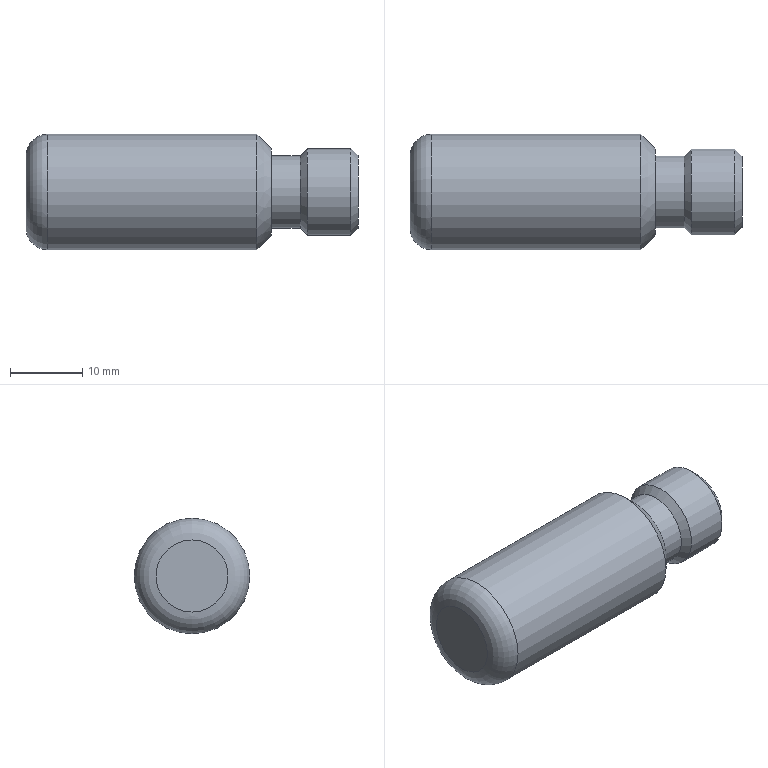Component | NX | ROCKER | 1 solid | 10 faces | volume 7838 mm3 | plane 3 | cylinder 3 | cone 3 | torus 1 | commonest cylinder face diameters 16 x1 10 x1 12 x1